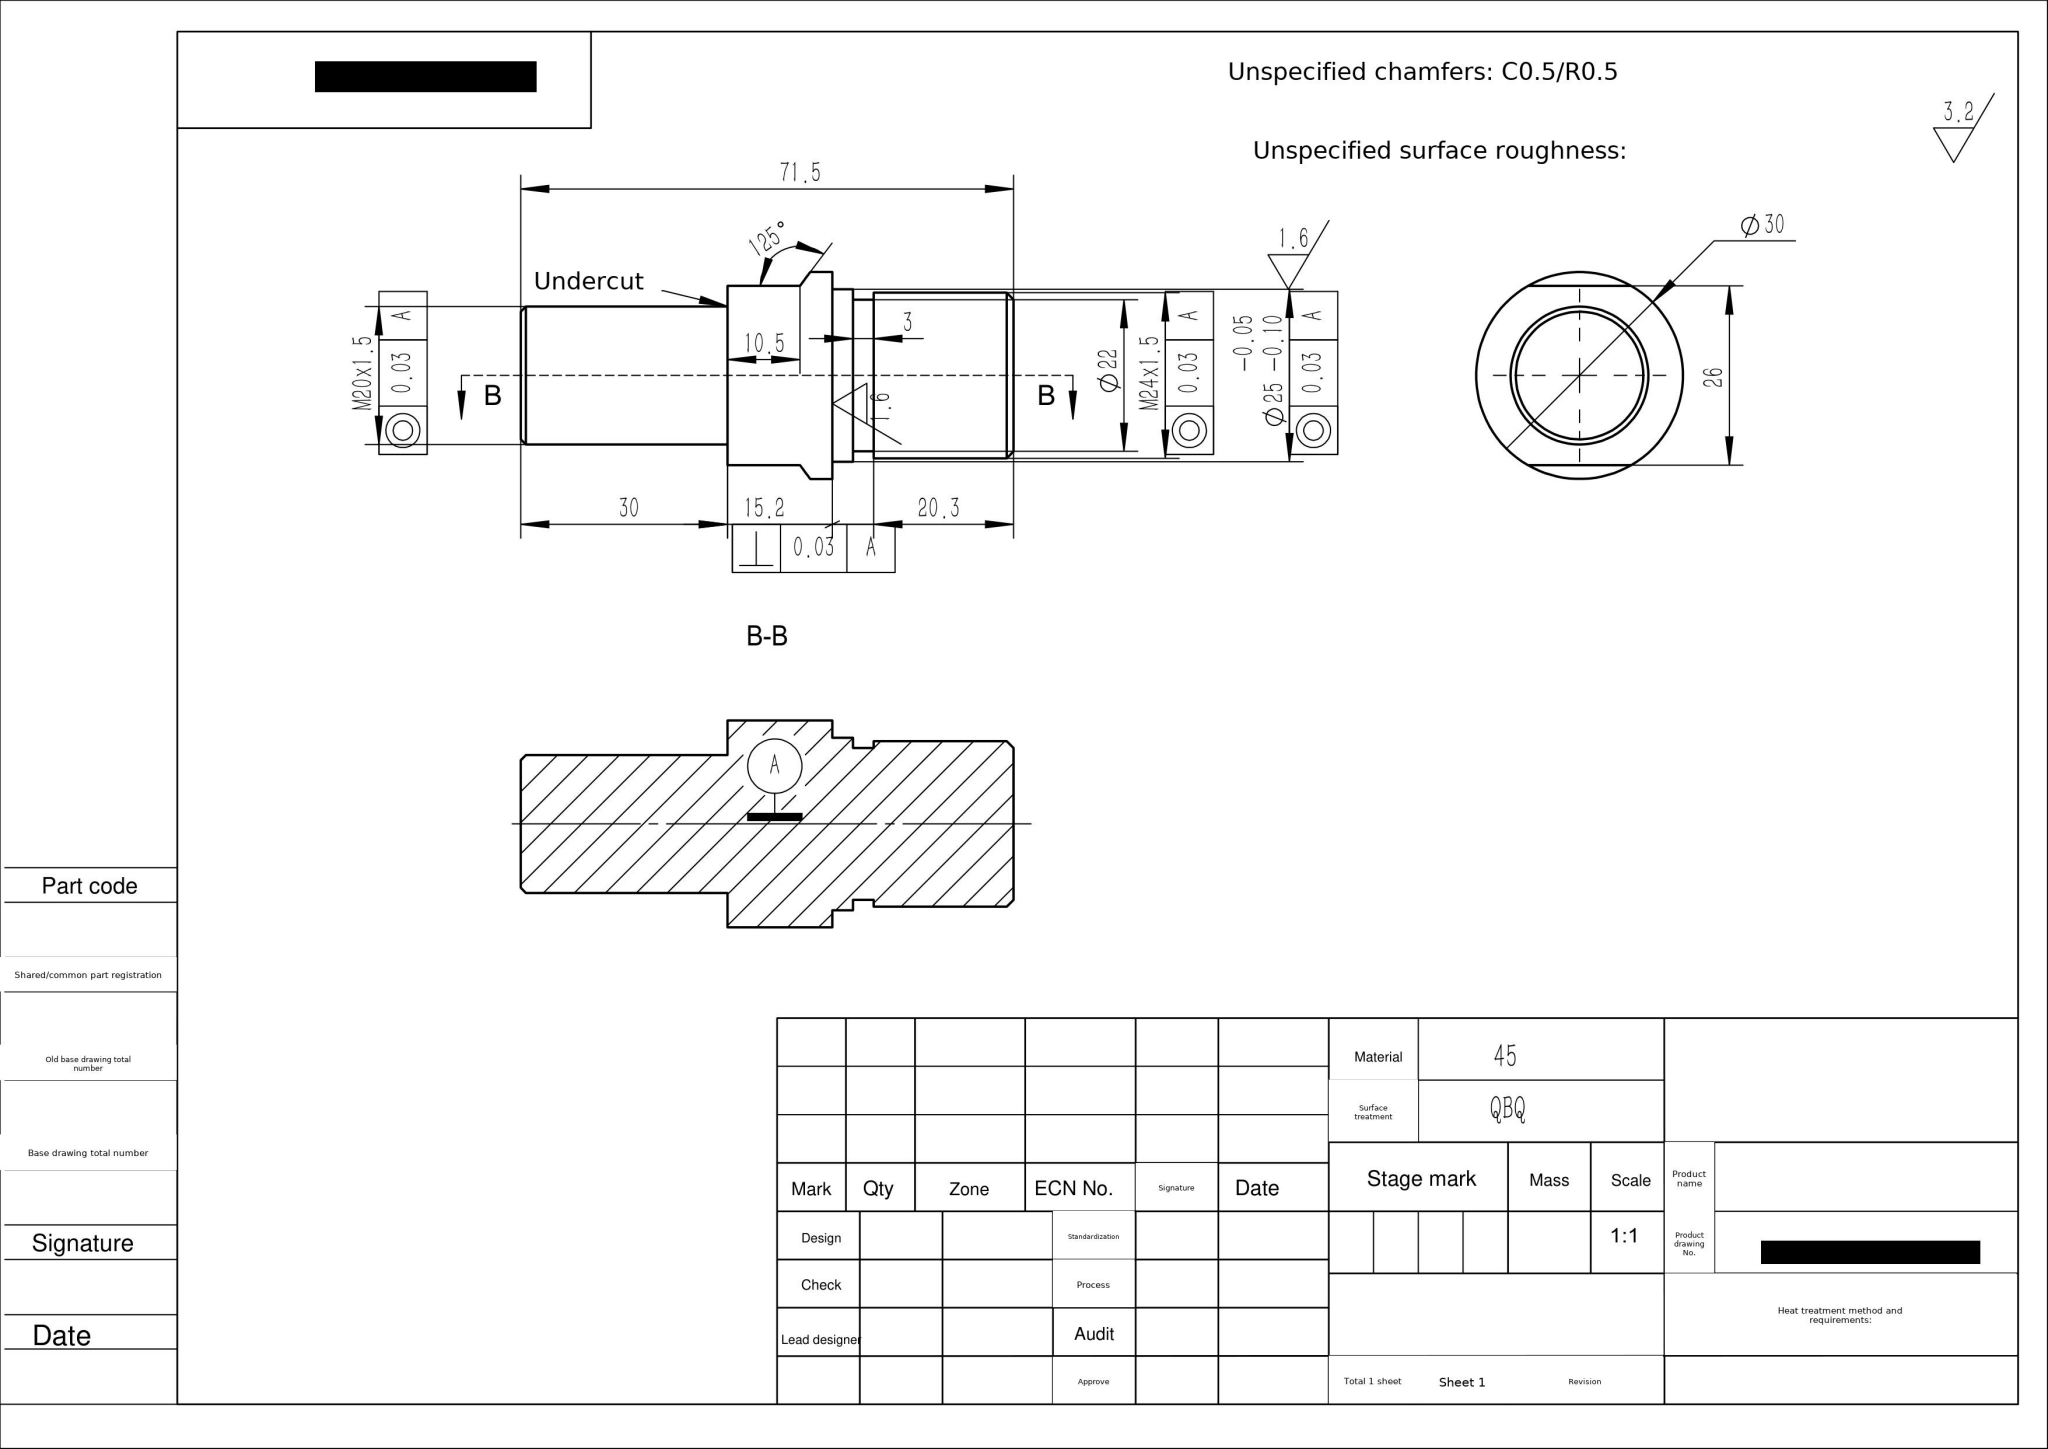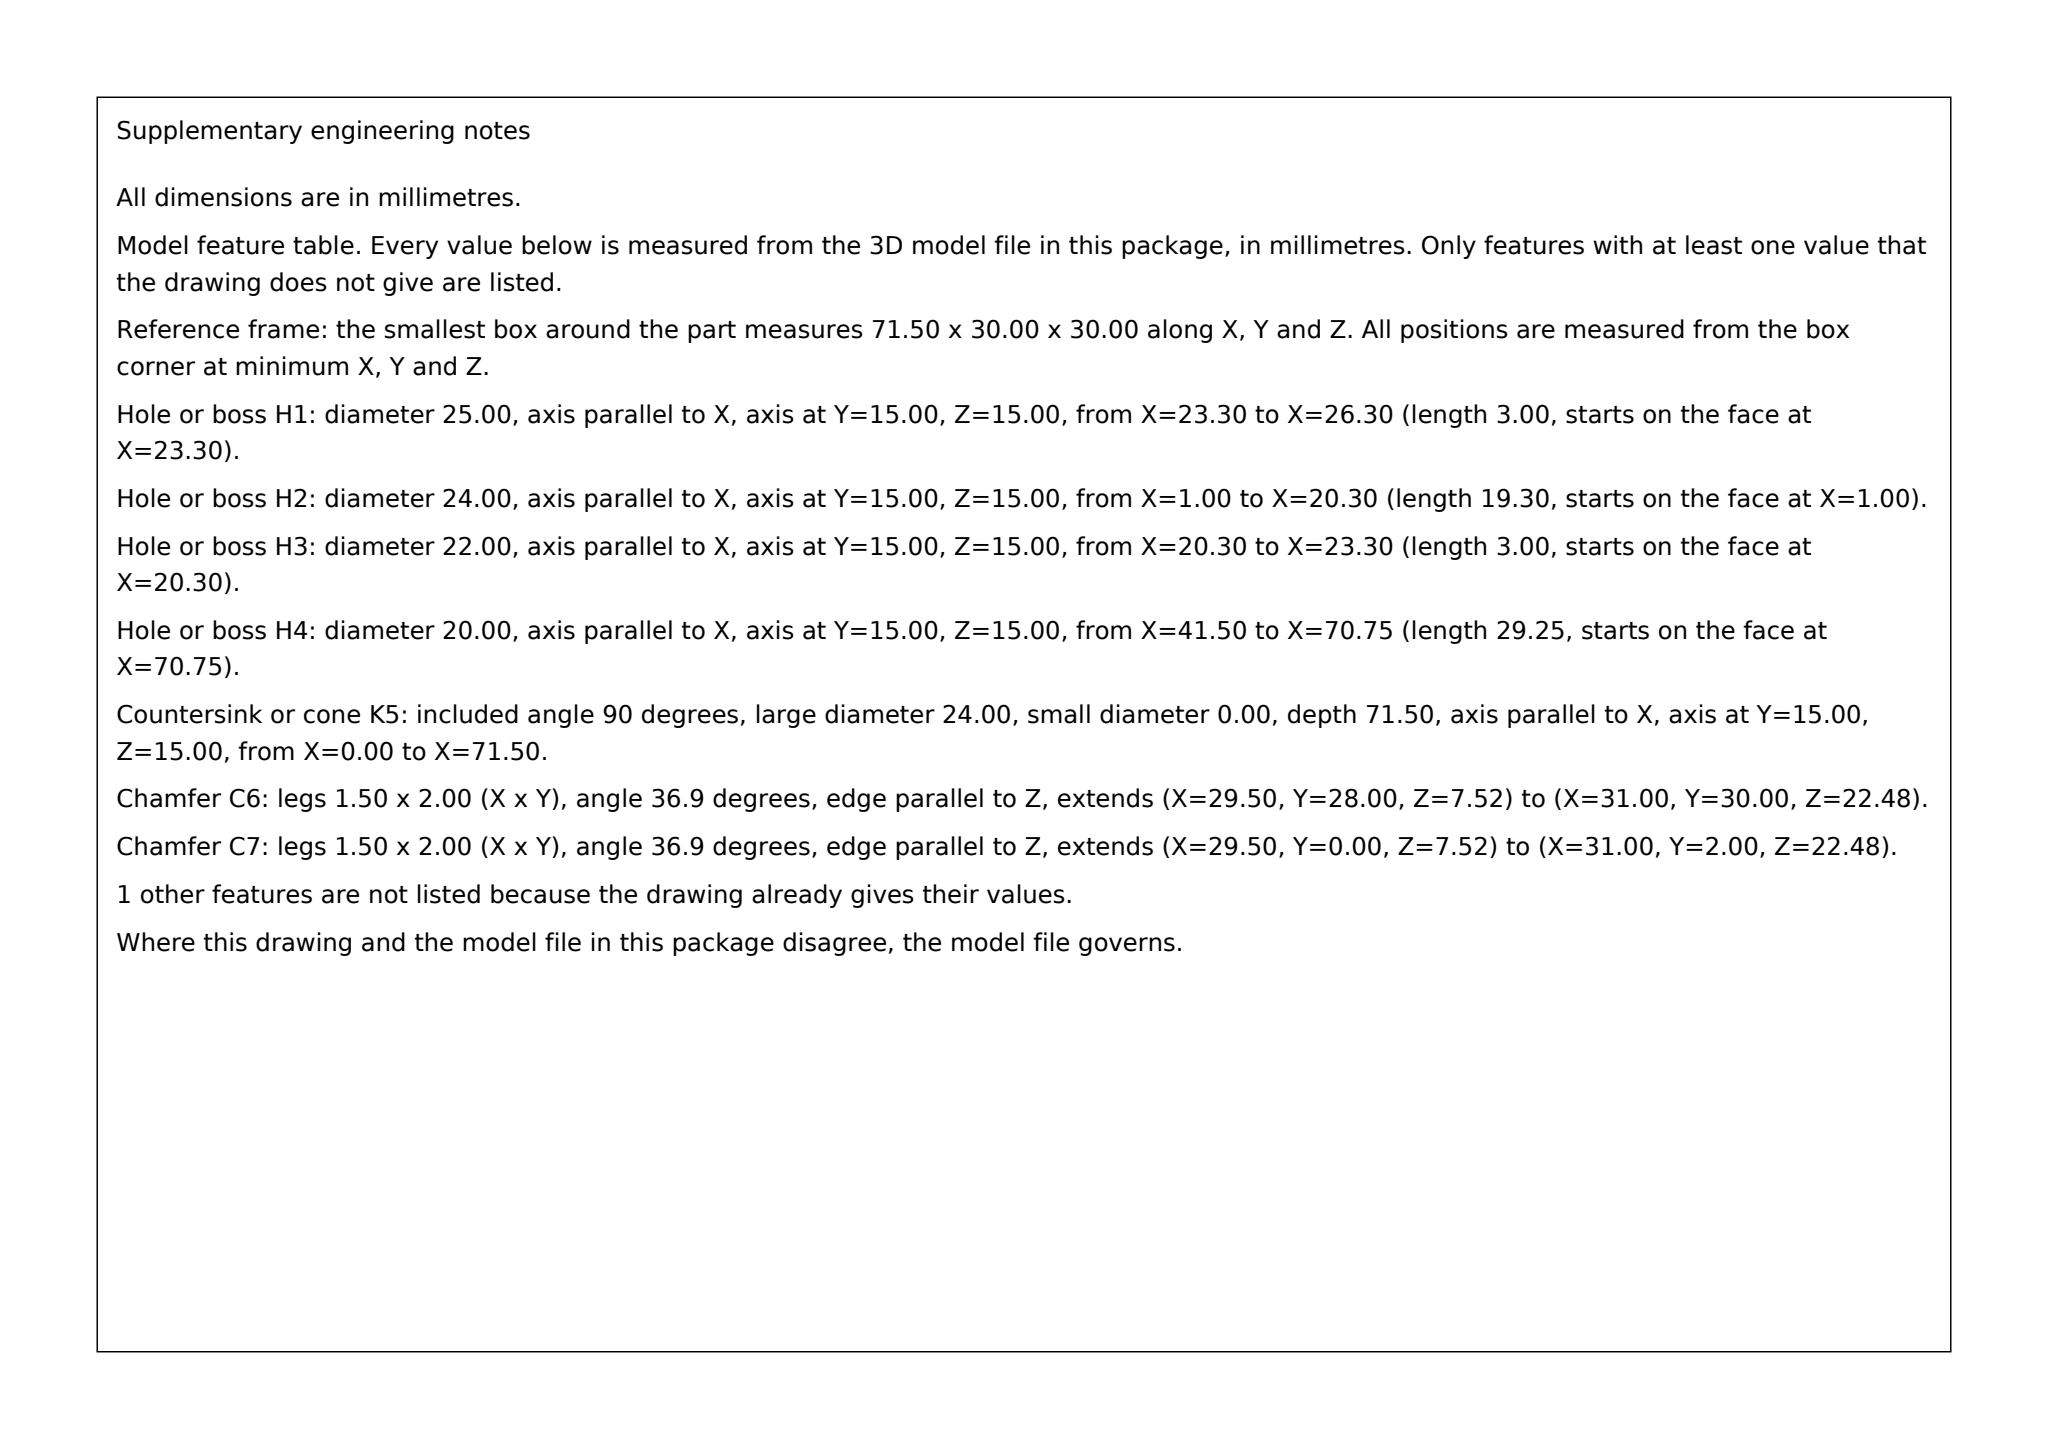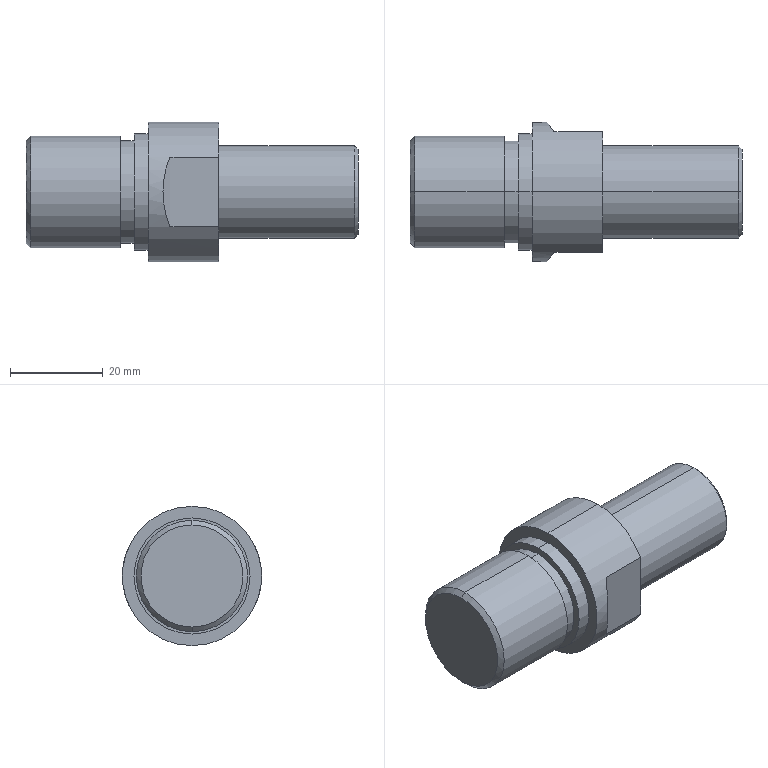Part | SolidWorks | mm | material 45 | 1 solid | 24 faces | box 71.5 x 30 x 30 mm | volume 31462 mm3 | cylinder 10 | plane 10 | cone 4 | commonest cylinder face diameters 20 x2 24 x2 22 x2 25 x2 30 x2
STEP:
#1=CARTESIAN_POINT('',(35.75,0.,-9.25));
#2=VERTEX_POINT('',#1);
#3=CARTESIAN_POINT('',(35.75,0.,9.25));
#4=VERTEX_POINT('',#3);
#5=CARTESIAN_POINT('',(35.75,0.,0.));
#6=DIRECTION('',(1.,0.,0.));
#7=DIRECTION('',(0.,0.,-1.));
#8=AXIS2_PLACEMENT_3D('',#5,#6,#7);
#9=CIRCLE('',#8,9.25);
#10=EDGE_CURVE('',#2,#4,#9,.T.);
#11=ORIENTED_EDGE('',*,*,#10,.F.);
#12=CARTESIAN_POINT('',(35.,0.,-10.));
#13=VERTEX_POINT('',#12);
#14=CARTESIAN_POINT('',(35.75,0.,-9.25));
#15=DIRECTION('',(-0.7071,0.,-0.7071));
#16=VECTOR('',#15,1000.);
#17=LINE('',#14,#16);
#18=EDGE_CURVE('',#2,#13,#17,.T.);
#19=ORIENTED_EDGE('',*,*,#18,.T.);
#20=CARTESIAN_POINT('',(35.,0.,10.));
#21=VERTEX_POINT('',#20);
#22=CARTESIAN_POINT('',(35.,0.,0.));
#23=DIRECTION('',(-1.,0.,0.));
#24=DIRECTION('',(0.,0.,-1.));
#25=AXIS2_PLACEMENT_3D('',#22,#23,#24);
#26=CIRCLE('',#25,10.);
#27=EDGE_CURVE('',#21,#13,#26,.T.);
#28=ORIENTED_EDGE('',*,*,#27,.F.);
#29=CARTESIAN_POINT('',(35.75,0.,9.25));
#30=DIRECTION('',(-0.7071,0.,0.7071));
#31=VECTOR('',#30,1000.);
#32=LINE('',#29,#31);
#33=EDGE_CURVE('',#4,#21,#32,.T.);
#34=ORIENTED_EDGE('',*,*,#33,.F.);
#35=EDGE_LOOP('',(#11,#19,#28,#34));
#36=FACE_OUTER_BOUND('',#35,.T.);
#37=CARTESIAN_POINT('',(35.75,0.,0.));
#38=DIRECTION('',(-1.,0.,0.));
#39=DIRECTION('',(0.,0.,1.));
#40=AXIS2_PLACEMENT_3D('',#37,#38,#39);
#41=CONICAL_SURFACE('',#40,9.25,0.7854);
#42=ADVANCED_FACE('',(#36),#41,.T.);
#43=ORIENTED_EDGE('',*,*,#27,.T.);
#44=CARTESIAN_POINT('',(5.75,0.,-10.));
#45=VERTEX_POINT('',#44);
#46=CARTESIAN_POINT('',(48.75,0.,-10.));
#47=DIRECTION('',(-1.,0.,0.));
#48=VECTOR('',#47,1000.);
#49=LINE('',#46,#48);
#50=EDGE_CURVE('',#13,#45,#49,.T.);
#51=ORIENTED_EDGE('',*,*,#50,.T.);
#52=CARTESIAN_POINT('',(5.75,0.,10.));
#53=VERTEX_POINT('',#52);
#54=CARTESIAN_POINT('',(5.75,0.,0.));
#55=DIRECTION('',(1.,0.,0.));
#56=DIRECTION('',(0.,0.,-1.));
#57=AXIS2_PLACEMENT_3D('',#54,#55,#56);
#58=CIRCLE('',#57,10.);
#59=EDGE_CURVE('',#45,#53,#58,.T.);
#60=ORIENTED_EDGE('',*,*,#59,.T.);
#61=CARTESIAN_POINT('',(48.75,0.,10.));
#62=DIRECTION('',(-1.,0.,0.));
#63=VECTOR('',#62,1000.);
#64=LINE('',#61,#63);
#65=EDGE_CURVE('',#21,#53,#64,.T.);
#66=ORIENTED_EDGE('',*,*,#65,.F.);
#67=EDGE_LOOP('',(#43,#51,#60,#66));
#68=FACE_OUTER_BOUND('',#67,.T.);
#69=CARTESIAN_POINT('',(48.75,0.,0.));
#70=DIRECTION('',(-1.,0.,0.));
#71=DIRECTION('',(0.,0.,1.));
#72=AXIS2_PLACEMENT_3D('',#69,#70,#71);
#73=CYLINDRICAL_SURFACE('',#72,10.);
#74=ADVANCED_FACE('',(#68),#73,.T.);
#75=CARTESIAN_POINT('',(-15.45,0.,-12.));
#76=VERTEX_POINT('',#75);
#77=CARTESIAN_POINT('',(-15.45,0.,12.));
#78=VERTEX_POINT('',#77);
#79=CARTESIAN_POINT('',(-15.45,0.,0.));
#80=DIRECTION('',(1.,0.,0.));
#81=DIRECTION('',(0.,0.,1.));
#82=AXIS2_PLACEMENT_3D('',#79,#80,#81);
#83=CIRCLE('',#82,12.);
#84=EDGE_CURVE('',#76,#78,#83,.T.);
#85=ORIENTED_EDGE('',*,*,#84,.F.);
#86=CARTESIAN_POINT('',(-34.75,0.,-12.));
#87=VERTEX_POINT('',#86);
#88=CARTESIAN_POINT('',(-11.75,0.,-12.));
#89=DIRECTION('',(-1.,0.,0.));
#90=VECTOR('',#89,1000.);
#91=LINE('',#88,#90);
#92=EDGE_CURVE('',#76,#87,#91,.T.);
#93=ORIENTED_EDGE('',*,*,#92,.T.);
#94=CARTESIAN_POINT('',(-34.75,0.,12.));
#95=VERTEX_POINT('',#94);
#96=CARTESIAN_POINT('',(-34.75,0.,0.));
#97=DIRECTION('',(1.,0.,0.));
#98=DIRECTION('',(0.,0.,1.));
#99=AXIS2_PLACEMENT_3D('',#96,#97,#98);
#100=CIRCLE('',#99,12.);
#101=EDGE_CURVE('',#87,#95,#100,.T.);
#102=ORIENTED_EDGE('',*,*,#101,.T.);
#103=CARTESIAN_POINT('',(-11.75,0.,12.));
#104=DIRECTION('',(-1.,0.,0.));
#105=VECTOR('',#104,1000.);
#106=LINE('',#103,#105);
#107=EDGE_CURVE('',#78,#95,#106,.T.);
#108=ORIENTED_EDGE('',*,*,#107,.F.);
#109=EDGE_LOOP('',(#85,#93,#102,#108));
#110=FACE_OUTER_BOUND('',#109,.T.);
#111=CARTESIAN_POINT('',(-11.75,0.,0.));
#112=DIRECTION('',(-1.,0.,0.));
#113=DIRECTION('',(0.,0.,1.));
#114=AXIS2_PLACEMENT_3D('',#111,#112,#113);
#115=CYLINDRICAL_SURFACE('',#114,12.);
#116=ADVANCED_FACE('',(#110),#115,.T.);
#117=CARTESIAN_POINT('',(-35.75,0.,-11.));
#118=VERTEX_POINT('',#117);
#119=CARTESIAN_POINT('',(-35.75,0.,11.));
#120=VERTEX_POINT('',#119);
#121=CARTESIAN_POINT('',(-35.75,0.,0.));
#122=DIRECTION('',(1.,0.,0.));
#123=DIRECTION('',(0.,0.,-1.));
#124=AXIS2_PLACEMENT_3D('',#121,#122,#123);
#125=CIRCLE('',#124,11.);
#126=EDGE_CURVE('',#118,#120,#125,.T.);
#127=ORIENTED_EDGE('',*,*,#126,.T.);
#128=CARTESIAN_POINT('',(-34.75,0.,12.));
#129=DIRECTION('',(0.7071,0.,0.7071));
#130=VECTOR('',#129,1000.);
#131=LINE('',#128,#130);
#132=EDGE_CURVE('',#120,#95,#131,.T.);
#133=ORIENTED_EDGE('',*,*,#132,.T.);
#134=ORIENTED_EDGE('',*,*,#101,.F.);
#135=CARTESIAN_POINT('',(-34.75,0.,-12.));
#136=DIRECTION('',(0.7071,0.,-0.7071));
#137=VECTOR('',#136,1000.);
#138=LINE('',#135,#137);
#139=EDGE_CURVE('',#118,#87,#138,.T.);
#140=ORIENTED_EDGE('',*,*,#139,.F.);
#141=EDGE_LOOP('',(#127,#133,#134,#140));
#142=FACE_OUTER_BOUND('',#141,.T.);
#143=CARTESIAN_POINT('',(-34.75,0.,0.));
#144=DIRECTION('',(1.,0.,0.));
#145=DIRECTION('',(0.,0.,-1.));
#146=AXIS2_PLACEMENT_3D('',#143,#144,#145);
#147=CONICAL_SURFACE('',#146,12.,0.7854);
#148=ADVANCED_FACE('',(#142),#147,.T.);
#149=CARTESIAN_POINT('',(-15.45,0.,11.));
#150=VERTEX_POINT('',#149);
#151=CARTESIAN_POINT('',(-15.45,0.,-11.));
#152=VERTEX_POINT('',#151);
#153=CARTESIAN_POINT('',(-15.45,0.,0.));
#154=DIRECTION('',(-1.,0.,0.));
#155=DIRECTION('',(0.,0.,1.));
#156=AXIS2_PLACEMENT_3D('',#153,#154,#155);
#157=CIRCLE('',#156,11.);
#158=EDGE_CURVE('',#150,#152,#157,.T.);
#159=ORIENTED_EDGE('',*,*,#158,.F.);
#160=CARTESIAN_POINT('',(-12.45,0.,11.));
#161=VERTEX_POINT('',#160);
#162=CARTESIAN_POINT('',(-15.45,0.,11.));
#163=DIRECTION('',(1.,0.,0.));
#164=VECTOR('',#163,1000.);
#165=LINE('',#162,#164);
#166=EDGE_CURVE('',#150,#161,#165,.T.);
#167=ORIENTED_EDGE('',*,*,#166,.T.);
#168=CARTESIAN_POINT('',(-12.45,0.,-11.));
#169=VERTEX_POINT('',#168);
#170=CARTESIAN_POINT('',(-12.45,0.,0.));
#171=DIRECTION('',(-1.,0.,0.));
#172=DIRECTION('',(0.,0.,1.));
#173=AXIS2_PLACEMENT_3D('',#170,#171,#172);
#174=CIRCLE('',#173,11.);
#175=EDGE_CURVE('',#161,#169,#174,.T.);
#176=ORIENTED_EDGE('',*,*,#175,.T.);
#177=CARTESIAN_POINT('',(-15.45,0.,-11.));
#178=DIRECTION('',(1.,0.,0.));
#179=VECTOR('',#178,1000.);
#180=LINE('',#177,#179);
#181=EDGE_CURVE('',#152,#169,#180,.T.);
#182=ORIENTED_EDGE('',*,*,#181,.F.);
#183=EDGE_LOOP('',(#159,#167,#176,#182));
#184=FACE_OUTER_BOUND('',#183,.T.);
#185=CARTESIAN_POINT('',(-15.45,0.,0.));
#186=DIRECTION('',(1.,0.,0.));
#187=DIRECTION('',(0.,0.,-1.));
#188=AXIS2_PLACEMENT_3D('',#185,#186,#187);
#189=CYLINDRICAL_SURFACE('',#188,11.);
#190=ADVANCED_FACE('',(#184),#189,.T.);
#191=CARTESIAN_POINT('',(-12.45,0.,12.5));
#192=VERTEX_POINT('',#191);
#193=CARTESIAN_POINT('',(-12.45,0.,-12.5));
#194=VERTEX_POINT('',#193);
#195=CARTESIAN_POINT('',(-12.45,0.,0.));
#196=DIRECTION('',(-1.,0.,0.));
#197=DIRECTION('',(0.,0.,1.));
#198=AXIS2_PLACEMENT_3D('',#195,#196,#197);
#199=CIRCLE('',#198,12.5);
#200=EDGE_CURVE('',#192,#194,#199,.T.);
#201=ORIENTED_EDGE('',*,*,#200,.F.);
#202=CARTESIAN_POINT('',(-9.45,0.,12.5));
#203=VERTEX_POINT('',#202);
#204=CARTESIAN_POINT('',(-35.75,0.,12.5));
#205=DIRECTION('',(1.,0.,0.));
#206=VECTOR('',#205,1000.);
#207=LINE('',#204,#206);
#208=EDGE_CURVE('',#192,#203,#207,.T.);
#209=ORIENTED_EDGE('',*,*,#208,.T.);
#210=CARTESIAN_POINT('',(-9.45,0.,-12.5));
#211=VERTEX_POINT('',#210);
#212=CARTESIAN_POINT('',(-9.45,0.,0.));
#213=DIRECTION('',(1.,0.,0.));
#214=DIRECTION('',(0.,0.,1.));
#215=AXIS2_PLACEMENT_3D('',#212,#213,#214);
#216=CIRCLE('',#215,12.5);
#217=EDGE_CURVE('',#211,#203,#216,.T.);
#218=ORIENTED_EDGE('',*,*,#217,.F.);
#219=CARTESIAN_POINT('',(-35.75,0.,-12.5));
#220=DIRECTION('',(1.,0.,0.));
#221=VECTOR('',#220,1000.);
#222=LINE('',#219,#221);
#223=EDGE_CURVE('',#194,#211,#222,.T.);
#224=ORIENTED_EDGE('',*,*,#223,.F.);
#225=EDGE_LOOP('',(#201,#209,#218,#224));
#226=FACE_OUTER_BOUND('',#225,.T.);
#227=CARTESIAN_POINT('',(-35.75,0.,0.));
#228=DIRECTION('',(1.,0.,0.));
#229=DIRECTION('',(0.,0.,-1.));
#230=AXIS2_PLACEMENT_3D('',#227,#228,#229);
#231=CYLINDRICAL_SURFACE('',#230,12.5);
#232=ADVANCED_FACE('',(#226),#231,.T.);
#233=CARTESIAN_POINT('',(5.75,0.,-15.));
#234=VERTEX_POINT('',#233);
#235=CARTESIAN_POINT('',(5.75,13.,-7.483));
#236=VERTEX_POINT('',#235);
#237=CARTESIAN_POINT('',(5.75,0.,0.));
#238=DIRECTION('',(1.,0.,0.));
#239=DIRECTION('',(0.,0.,1.));
#240=AXIS2_PLACEMENT_3D('',#237,#238,#239);
#241=CIRCLE('',#240,15.);
#242=EDGE_CURVE('',#234,#236,#241,.T.);
#243=ORIENTED_EDGE('',*,*,#242,.F.);
#244=CARTESIAN_POINT('',(-9.45,0.,-15.));
#245=VERTEX_POINT('',#244);
#246=CARTESIAN_POINT('',(8.75,0.,-15.));
#247=DIRECTION('',(-1.,0.,0.));
#248=VECTOR('',#247,1000.);
#249=LINE('',#246,#248);
#250=EDGE_CURVE('',#234,#245,#249,.T.);
#251=ORIENTED_EDGE('',*,*,#250,.T.);
#252=CARTESIAN_POINT('',(-9.45,0.,15.));
#253=VERTEX_POINT('',#252);
#254=CARTESIAN_POINT('',(-9.45,0.,0.));
#255=DIRECTION('',(-1.,0.,0.));
#256=DIRECTION('',(0.,0.,1.));
#257=AXIS2_PLACEMENT_3D('',#254,#255,#256);
#258=CIRCLE('',#257,15.);
#259=EDGE_CURVE('',#253,#245,#258,.T.);
#260=ORIENTED_EDGE('',*,*,#259,.F.);
#261=CARTESIAN_POINT('',(5.75,0.,15.));
#262=VERTEX_POINT('',#261);
#263=CARTESIAN_POINT('',(8.75,0.,15.));
#264=DIRECTION('',(-1.,0.,0.));
#265=VECTOR('',#264,1000.);
#266=LINE('',#263,#265);
#267=EDGE_CURVE('',#262,#253,#266,.T.);
#268=ORIENTED_EDGE('',*,*,#267,.F.);
#269=CARTESIAN_POINT('',(5.75,13.,7.483));
#270=VERTEX_POINT('',#269);
#271=CARTESIAN_POINT('',(5.75,0.,0.));
#272=DIRECTION('',(1.,0.,0.));
#273=DIRECTION('',(0.,0.,1.));
#274=AXIS2_PLACEMENT_3D('',#271,#272,#273);
#275=CIRCLE('',#274,15.);
#276=EDGE_CURVE('',#270,#262,#275,.T.);
#277=ORIENTED_EDGE('',*,*,#276,.F.);
#278=CARTESIAN_POINT('',(-4.75,13.,7.483));
#279=VERTEX_POINT('',#278);
#280=CARTESIAN_POINT('',(-4.75,13.,7.483));
#281=DIRECTION('',(1.,0.,0.));
#282=VECTOR('',#281,1000.);
#283=LINE('',#280,#282);
#284=EDGE_CURVE('',#279,#270,#283,.T.);
#285=ORIENTED_EDGE('',*,*,#284,.F.);
#286=CARTESIAN_POINT('',(-4.75,13.,-7.483));
#287=VERTEX_POINT('',#286);
#288=CARTESIAN_POINT('',(-4.75,13.,7.483));
#289=CARTESIAN_POINT('',(-6.799,15.732,2.738));
#290=CARTESIAN_POINT('',(-6.799,15.732,-2.738));
#291=CARTESIAN_POINT('',(-4.75,13.,-7.483));
#292=(BOUNDED_CURVE()B_SPLINE_CURVE(3,(#288,#289,#290,#291),.UNSPECIFIED.,.F.,.T.)B_SPLINE_CURVE_WITH_KNOTS((4,4),(5.761,6.806),.UNSPECIFIED.)CURVE()GEOMETRIC_REPRESENTATION_ITEM()RATIONAL_B_SPLINE_CURVE((1.,0.9111,0.9111,1.))REPRESENTATION_ITEM(''));
#293=EDGE_CURVE('',#279,#287,#292,.T.);
#294=ORIENTED_EDGE('',*,*,#293,.T.);
#295=CARTESIAN_POINT('',(-4.75,13.,-7.483));
#296=DIRECTION('',(-1.,0.,0.));
#297=VECTOR('',#296,1000.);
#298=LINE('',#295,#297);
#299=EDGE_CURVE('',#236,#287,#298,.T.);
#300=ORIENTED_EDGE('',*,*,#299,.F.);
#301=EDGE_LOOP('',(#243,#251,#260,#268,#277,#285,#294,#300));
#302=FACE_OUTER_BOUND('',#301,.T.);
#303=CARTESIAN_POINT('',(8.75,0.,0.));
#304=DIRECTION('',(-1.,0.,0.));
#305=DIRECTION('',(0.,0.,1.));
#306=AXIS2_PLACEMENT_3D('',#303,#304,#305);
#307=CYLINDRICAL_SURFACE('',#306,15.);
#308=ADVANCED_FACE('',(#302),#307,.T.);
#309=CARTESIAN_POINT('',(5.75,0.,0.));
#310=DIRECTION('',(1.,0.,0.));
#311=DIRECTION('',(0.,0.,-1.));
#312=AXIS2_PLACEMENT_3D('',#309,#310,#311);
#313=CIRCLE('',#312,10.);
#314=EDGE_CURVE('',#53,#45,#313,.T.);
#315=ORIENTED_EDGE('',*,*,#314,.F.);
#316=ORIENTED_EDGE('',*,*,#59,.F.);
#317=EDGE_LOOP('',(#315,#316));
#318=FACE_BOUND('',#317,.T.);
#319=CARTESIAN_POINT('',(5.75,-13.,-7.483));
#320=VERTEX_POINT('',#319);
#321=CARTESIAN_POINT('',(5.75,0.,0.));
#322=DIRECTION('',(1.,0.,0.));
#323=DIRECTION('',(0.,0.,1.));
#324=AXIS2_PLACEMENT_3D('',#321,#322,#323);
#325=CIRCLE('',#324,15.);
#326=EDGE_CURVE('',#320,#234,#325,.T.);
#327=ORIENTED_EDGE('',*,*,#326,.T.);
#328=ORIENTED_EDGE('',*,*,#242,.T.);
#329=CARTESIAN_POINT('',(5.75,13.,0.));
#330=DIRECTION('',(0.,0.,1.));
#331=VECTOR('',#330,1000.);
#332=LINE('',#329,#331);
#333=EDGE_CURVE('',#236,#270,#332,.T.);
#334=ORIENTED_EDGE('',*,*,#333,.T.);
#335=ORIENTED_EDGE('',*,*,#276,.T.);
#336=CARTESIAN_POINT('',(5.75,-13.,7.483));
#337=VERTEX_POINT('',#336);
#338=CARTESIAN_POINT('',(5.75,0.,0.));
#339=DIRECTION('',(1.,0.,0.));
#340=DIRECTION('',(0.,0.,1.));
#341=AXIS2_PLACEMENT_3D('',#338,#339,#340);
#342=CIRCLE('',#341,15.);
#343=EDGE_CURVE('',#262,#337,#342,.T.);
#344=ORIENTED_EDGE('',*,*,#343,.T.);
#345=CARTESIAN_POINT('',(5.75,-13.,0.));
#346=DIRECTION('',(0.,0.,-1.));
#347=VECTOR('',#346,1000.);
#348=LINE('',#345,#347);
#349=EDGE_CURVE('',#337,#320,#348,.T.);
#350=ORIENTED_EDGE('',*,*,#349,.T.);
#351=EDGE_LOOP('',(#327,#328,#334,#335,#344,#350));
#352=FACE_OUTER_BOUND('',#351,.T.);
#353=CARTESIAN_POINT('',(5.75,0.,0.));
#354=DIRECTION('',(1.,0.,0.));
#355=DIRECTION('',(0.,0.,-1.));
#356=AXIS2_PLACEMENT_3D('',#353,#354,#355);
#357=PLANE('',#356);
#358=ADVANCED_FACE('',(#318,#352),#357,.T.);
#359=ORIENTED_EDGE('',*,*,#284,.T.);
#360=ORIENTED_EDGE('',*,*,#333,.F.);
#361=ORIENTED_EDGE('',*,*,#299,.T.);
#362=CARTESIAN_POINT('',(-4.75,13.,21.671));
#363=DIRECTION('',(0.,0.,1.));
#364=VECTOR('',#363,1000.);
#365=LINE('',#362,#364);
#366=EDGE_CURVE('',#287,#279,#365,.T.);
#367=ORIENTED_EDGE('',*,*,#366,.T.);
#368=EDGE_LOOP('',(#359,#360,#361,#367));
#369=FACE_OUTER_BOUND('',#368,.T.);
#370=CARTESIAN_POINT('',(-4.75,13.,21.671));
#371=DIRECTION('',(0.,1.,0.));
#372=DIRECTION('',(0.,0.,1.));
#373=AXIS2_PLACEMENT_3D('',#370,#371,#372);
#374=PLANE('',#373);
#375=ADVANCED_FACE('',(#369),#374,.T.);
#376=ORIENTED_EDGE('',*,*,#250,.F.);
#377=ORIENTED_EDGE('',*,*,#326,.F.);
#378=CARTESIAN_POINT('',(-4.75,-13.,-7.483));
#379=VERTEX_POINT('',#378);
#380=CARTESIAN_POINT('',(8.75,-13.,-7.483));
#381=DIRECTION('',(-1.,0.,0.));
#382=VECTOR('',#381,1000.);
#383=LINE('',#380,#382);
#384=EDGE_CURVE('',#320,#379,#383,.T.);
#385=ORIENTED_EDGE('',*,*,#384,.T.);
#386=CARTESIAN_POINT('',(-4.75,-13.,7.483));
#387=VERTEX_POINT('',#386);
#388=CARTESIAN_POINT('',(-4.75,-13.,-7.483));
#389=CARTESIAN_POINT('',(-6.799,-15.732,-2.738));
#390=CARTESIAN_POINT('',(-6.799,-15.732,2.738));
#391=CARTESIAN_POINT('',(-4.75,-13.,7.483));
#392=(BOUNDED_CURVE()B_SPLINE_CURVE(3,(#388,#389,#390,#391),.UNSPECIFIED.,.F.,.F.)B_SPLINE_CURVE_WITH_KNOTS((4,4),(5.761,6.806),.UNSPECIFIED.)CURVE()GEOMETRIC_REPRESENTATION_ITEM()RATIONAL_B_SPLINE_CURVE((1.,0.9111,0.9111,1.))REPRESENTATION_ITEM(''));
#393=EDGE_CURVE('',#379,#387,#392,.T.);
#394=ORIENTED_EDGE('',*,*,#393,.T.);
#395=CARTESIAN_POINT('',(8.75,-13.,7.483));
#396=DIRECTION('',(1.,0.,0.));
#397=VECTOR('',#396,1000.);
#398=LINE('',#395,#397);
#399=EDGE_CURVE('',#387,#337,#398,.T.);
#400=ORIENTED_EDGE('',*,*,#399,.T.);
#401=ORIENTED_EDGE('',*,*,#343,.F.);
#402=ORIENTED_EDGE('',*,*,#267,.T.);
#403=CARTESIAN_POINT('',(-9.45,0.,0.));
#404=DIRECTION('',(-1.,0.,0.));
#405=DIRECTION('',(0.,0.,1.));
#406=AXIS2_PLACEMENT_3D('',#403,#404,#405);
#407=CIRCLE('',#406,15.);
#408=EDGE_CURVE('',#245,#253,#407,.T.);
#409=ORIENTED_EDGE('',*,*,#408,.F.);
#410=EDGE_LOOP('',(#376,#377,#385,#394,#400,#401,#402,#409));
#411=FACE_OUTER_BOUND('',#410,.T.);
#412=CARTESIAN_POINT('',(8.75,0.,0.));
#413=DIRECTION('',(-1.,0.,0.));
#414=DIRECTION('',(0.,0.,1.));
#415=AXIS2_PLACEMENT_3D('',#412,#413,#414);
#416=CYLINDRICAL_SURFACE('',#415,15.);
#417=ADVANCED_FACE('',(#411),#416,.T.);
#418=ORIENTED_EDGE('',*,*,#384,.F.);
#419=ORIENTED_EDGE('',*,*,#349,.F.);
#420=ORIENTED_EDGE('',*,*,#399,.F.);
#421=CARTESIAN_POINT('',(-4.75,-13.,21.671));
#422=DIRECTION('',(0.,0.,-1.));
#423=VECTOR('',#422,1000.);
#424=LINE('',#421,#423);
#425=EDGE_CURVE('',#387,#379,#424,.T.);
#426=ORIENTED_EDGE('',*,*,#425,.T.);
#427=EDGE_LOOP('',(#418,#419,#420,#426));
#428=FACE_OUTER_BOUND('',#427,.T.);
#429=CARTESIAN_POINT('',(-4.75,-13.,21.671));
#430=DIRECTION('',(0.,-1.,0.));
#431=DIRECTION('',(0.,0.,-1.));
#432=AXIS2_PLACEMENT_3D('',#429,#430,#431);
#433=PLANE('',#432);
#434=ADVANCED_FACE('',(#428),#433,.T.);
#435=ORIENTED_EDGE('',*,*,#366,.F.);
#436=ORIENTED_EDGE('',*,*,#293,.F.);
#437=EDGE_LOOP('',(#435,#436));
#438=FACE_OUTER_BOUND('',#437,.T.);
#439=CARTESIAN_POINT('',(-4.75,13.,-15.));
#440=DIRECTION('',(-0.8,-0.6,0.));
#441=DIRECTION('',(0.6,-0.8,0.));
#442=AXIS2_PLACEMENT_3D('',#439,#440,#441);
#443=PLANE('',#442);
#444=ADVANCED_FACE('',(#438),#443,.F.);
#445=ORIENTED_EDGE('',*,*,#393,.F.);
#446=ORIENTED_EDGE('',*,*,#425,.F.);
#447=EDGE_LOOP('',(#445,#446));
#448=FACE_OUTER_BOUND('',#447,.T.);
#449=CARTESIAN_POINT('',(-4.75,-13.,-15.));
#450=DIRECTION('',(0.8,-0.6,0.));
#451=DIRECTION('',(0.6,0.8,0.));
#452=AXIS2_PLACEMENT_3D('',#449,#450,#451);
#453=PLANE('',#452);
#454=ADVANCED_FACE('',(#448),#453,.T.);
#455=ORIENTED_EDGE('',*,*,#259,.T.);
#456=ORIENTED_EDGE('',*,*,#408,.T.);
#457=EDGE_LOOP('',(#455,#456));
#458=FACE_OUTER_BOUND('',#457,.T.);
#459=ORIENTED_EDGE('',*,*,#217,.T.);
#460=CARTESIAN_POINT('',(-9.45,0.,0.));
#461=DIRECTION('',(1.,0.,0.));
#462=DIRECTION('',(0.,0.,1.));
#463=AXIS2_PLACEMENT_3D('',#460,#461,#462);
#464=CIRCLE('',#463,12.5);
#465=EDGE_CURVE('',#203,#211,#464,.T.);
#466=ORIENTED_EDGE('',*,*,#465,.T.);
#467=EDGE_LOOP('',(#459,#466));
#468=FACE_BOUND('',#467,.T.);
#469=CARTESIAN_POINT('',(-9.45,0.,0.));
#470=DIRECTION('',(-1.,0.,0.));
#471=DIRECTION('',(0.,0.,1.));
#472=AXIS2_PLACEMENT_3D('',#469,#470,#471);
#473=PLANE('',#472);
#474=ADVANCED_FACE('',(#458,#468),#473,.T.);
#475=ORIENTED_EDGE('',*,*,#208,.F.);
#476=CARTESIAN_POINT('',(-12.45,0.,0.));
#477=DIRECTION('',(-1.,0.,0.));
#478=DIRECTION('',(0.,0.,1.));
#479=AXIS2_PLACEMENT_3D('',#476,#477,#478);
#480=CIRCLE('',#479,12.5);
#481=EDGE_CURVE('',#194,#192,#480,.T.);
#482=ORIENTED_EDGE('',*,*,#481,.F.);
#483=ORIENTED_EDGE('',*,*,#223,.T.);
#484=ORIENTED_EDGE('',*,*,#465,.F.);
#485=EDGE_LOOP('',(#475,#482,#483,#484));
#486=FACE_OUTER_BOUND('',#485,.T.);
#487=CARTESIAN_POINT('',(-35.75,0.,0.));
#488=DIRECTION('',(1.,0.,0.));
#489=DIRECTION('',(0.,0.,-1.));
#490=AXIS2_PLACEMENT_3D('',#487,#488,#489);
#491=CYLINDRICAL_SURFACE('',#490,12.5);
#492=ADVANCED_FACE('',(#486),#491,.T.);
#493=ORIENTED_EDGE('',*,*,#481,.T.);
#494=ORIENTED_EDGE('',*,*,#200,.T.);
#495=EDGE_LOOP('',(#493,#494));
#496=FACE_OUTER_BOUND('',#495,.T.);
#497=CARTESIAN_POINT('',(-12.45,0.,0.));
#498=DIRECTION('',(-1.,0.,0.));
#499=DIRECTION('',(0.,0.,1.));
#500=AXIS2_PLACEMENT_3D('',#497,#498,#499);
#501=CIRCLE('',#500,11.);
#502=EDGE_CURVE('',#169,#161,#501,.T.);
#503=ORIENTED_EDGE('',*,*,#502,.F.);
#504=ORIENTED_EDGE('',*,*,#175,.F.);
#505=EDGE_LOOP('',(#503,#504));
#506=FACE_BOUND('',#505,.T.);
#507=CARTESIAN_POINT('',(-12.45,0.,0.));
#508=DIRECTION('',(-1.,0.,0.));
#509=DIRECTION('',(0.,0.,1.));
#510=AXIS2_PLACEMENT_3D('',#507,#508,#509);
#511=PLANE('',#510);
#512=ADVANCED_FACE('',(#496,#506),#511,.T.);
#513=CARTESIAN_POINT('',(-15.45,0.,0.));
#514=DIRECTION('',(1.,0.,0.));
#515=DIRECTION('',(0.,0.,1.));
#516=AXIS2_PLACEMENT_3D('',#513,#514,#515);
#517=CIRCLE('',#516,12.);
#518=EDGE_CURVE('',#78,#76,#517,.T.);
#519=ORIENTED_EDGE('',*,*,#518,.T.);
#520=ORIENTED_EDGE('',*,*,#84,.T.);
#521=EDGE_LOOP('',(#519,#520));
#522=FACE_OUTER_BOUND('',#521,.T.);
#523=CARTESIAN_POINT('',(-15.45,0.,0.));
#524=DIRECTION('',(-1.,0.,0.));
#525=DIRECTION('',(0.,0.,1.));
#526=AXIS2_PLACEMENT_3D('',#523,#524,#525);
#527=CIRCLE('',#526,11.);
#528=EDGE_CURVE('',#152,#150,#527,.T.);
#529=ORIENTED_EDGE('',*,*,#528,.T.);
#530=ORIENTED_EDGE('',*,*,#158,.T.);
#531=EDGE_LOOP('',(#529,#530));
#532=FACE_BOUND('',#531,.T.);
#533=CARTESIAN_POINT('',(-15.45,0.,0.));
#534=DIRECTION('',(-1.,0.,0.));
#535=DIRECTION('',(0.,0.,1.));
#536=AXIS2_PLACEMENT_3D('',#533,#534,#535);
#537=PLANE('',#536);
#538=ADVANCED_FACE('',(#522,#532),#537,.F.);
#539=ORIENTED_EDGE('',*,*,#166,.F.);
#540=ORIENTED_EDGE('',*,*,#528,.F.);
#541=ORIENTED_EDGE('',*,*,#181,.T.);
#542=ORIENTED_EDGE('',*,*,#502,.T.);
#543=EDGE_LOOP('',(#539,#540,#541,#542));
#544=FACE_OUTER_BOUND('',#543,.T.);
#545=CARTESIAN_POINT('',(-15.45,0.,0.));
#546=DIRECTION('',(1.,0.,0.));
#547=DIRECTION('',(0.,0.,-1.));
#548=AXIS2_PLACEMENT_3D('',#545,#546,#547);
#549=CYLINDRICAL_SURFACE('',#548,11.);
#550=ADVANCED_FACE('',(#544),#549,.T.);
#551=ORIENTED_EDGE('',*,*,#126,.F.);
#552=CARTESIAN_POINT('',(-35.75,0.,0.));
#553=DIRECTION('',(1.,0.,0.));
#554=DIRECTION('',(0.,0.,-1.));
#555=AXIS2_PLACEMENT_3D('',#552,#553,#554);
#556=CIRCLE('',#555,11.);
#557=EDGE_CURVE('',#120,#118,#556,.T.);
#558=ORIENTED_EDGE('',*,*,#557,.F.);
#559=EDGE_LOOP('',(#551,#558));
#560=FACE_OUTER_BOUND('',#559,.T.);
#561=CARTESIAN_POINT('',(-35.75,0.,0.));
#562=DIRECTION('',(-1.,0.,0.));
#563=DIRECTION('',(0.,0.,1.));
#564=AXIS2_PLACEMENT_3D('',#561,#562,#563);
#565=PLANE('',#564);
#566=ADVANCED_FACE('',(#560),#565,.T.);
#567=ORIENTED_EDGE('',*,*,#132,.F.);
#568=ORIENTED_EDGE('',*,*,#557,.T.);
#569=ORIENTED_EDGE('',*,*,#139,.T.);
#570=CARTESIAN_POINT('',(-34.75,0.,0.));
#571=DIRECTION('',(1.,0.,0.));
#572=DIRECTION('',(0.,0.,1.));
#573=AXIS2_PLACEMENT_3D('',#570,#571,#572);
#574=CIRCLE('',#573,12.);
#575=EDGE_CURVE('',#95,#87,#574,.T.);
#576=ORIENTED_EDGE('',*,*,#575,.F.);
#577=EDGE_LOOP('',(#567,#568,#569,#576));
#578=FACE_OUTER_BOUND('',#577,.T.);
#579=CARTESIAN_POINT('',(-34.75,0.,0.));
#580=DIRECTION('',(1.,0.,0.));
#581=DIRECTION('',(0.,0.,-1.));
#582=AXIS2_PLACEMENT_3D('',#579,#580,#581);
#583=CONICAL_SURFACE('',#582,12.,0.7854);
#584=ADVANCED_FACE('',(#578),#583,.T.);
#585=ORIENTED_EDGE('',*,*,#92,.F.);
#586=ORIENTED_EDGE('',*,*,#518,.F.);
#587=ORIENTED_EDGE('',*,*,#107,.T.);
#588=ORIENTED_EDGE('',*,*,#575,.T.);
#589=EDGE_LOOP('',(#585,#586,#587,#588));
#590=FACE_OUTER_BOUND('',#589,.T.);
#591=CARTESIAN_POINT('',(-11.75,0.,0.));
#592=DIRECTION('',(-1.,0.,0.));
#593=DIRECTION('',(0.,0.,1.));
#594=AXIS2_PLACEMENT_3D('',#591,#592,#593);
#595=CYLINDRICAL_SURFACE('',#594,12.);
#596=ADVANCED_FACE('',(#590),#595,.T.);
#597=ORIENTED_EDGE('',*,*,#50,.F.);
#598=CARTESIAN_POINT('',(35.,0.,0.));
#599=DIRECTION('',(-1.,0.,0.));
#600=DIRECTION('',(0.,0.,-1.));
#601=AXIS2_PLACEMENT_3D('',#598,#599,#600);
#602=CIRCLE('',#601,10.);
#603=EDGE_CURVE('',#13,#21,#602,.T.);
#604=ORIENTED_EDGE('',*,*,#603,.T.);
#605=ORIENTED_EDGE('',*,*,#65,.T.);
#606=ORIENTED_EDGE('',*,*,#314,.T.);
#607=EDGE_LOOP('',(#597,#604,#605,#606));
#608=FACE_OUTER_BOUND('',#607,.T.);
#609=CARTESIAN_POINT('',(48.75,0.,0.));
#610=DIRECTION('',(-1.,0.,0.));
#611=DIRECTION('',(0.,0.,1.));
#612=AXIS2_PLACEMENT_3D('',#609,#610,#611);
#613=CYLINDRICAL_SURFACE('',#612,10.);
#614=ADVANCED_FACE('',(#608),#613,.T.);
#615=CARTESIAN_POINT('',(35.75,0.,0.));
#616=DIRECTION('',(1.,0.,0.));
#617=DIRECTION('',(0.,0.,-1.));
#618=AXIS2_PLACEMENT_3D('',#615,#616,#617);
#619=CIRCLE('',#618,9.25);
#620=EDGE_CURVE('',#4,#2,#619,.T.);
#621=ORIENTED_EDGE('',*,*,#620,.T.);
#622=ORIENTED_EDGE('',*,*,#10,.T.);
#623=EDGE_LOOP('',(#621,#622));
#624=FACE_OUTER_BOUND('',#623,.T.);
#625=CARTESIAN_POINT('',(35.75,0.,0.));
#626=DIRECTION('',(1.,0.,0.));
#627=DIRECTION('',(0.,0.,-1.));
#628=AXIS2_PLACEMENT_3D('',#625,#626,#627);
#629=PLANE('',#628);
#630=ADVANCED_FACE('',(#624),#629,.T.);
#631=ORIENTED_EDGE('',*,*,#18,.F.);
#632=ORIENTED_EDGE('',*,*,#620,.F.);
#633=ORIENTED_EDGE('',*,*,#33,.T.);
#634=ORIENTED_EDGE('',*,*,#603,.F.);
#635=EDGE_LOOP('',(#631,#632,#633,#634));
#636=FACE_OUTER_BOUND('',#635,.T.);
#637=CARTESIAN_POINT('',(35.75,0.,0.));
#638=DIRECTION('',(-1.,0.,0.));
#639=DIRECTION('',(0.,0.,1.));
#640=AXIS2_PLACEMENT_3D('',#637,#638,#639);
#641=CONICAL_SURFACE('',#640,9.25,0.7854);
#642=ADVANCED_FACE('',(#636),#641,.T.);
#643=CLOSED_SHELL('',(#42,#74,#116,#148,#190,#232,#308,#358,#375,#417,#434,#444,#454,#474,#492,#512,#538,#550,#566,#584,#596,#614,#630,#642));
#644=MANIFOLD_SOLID_BREP('',#643);
#645=CARTESIAN_POINT('',(0.,0.,0.));
#646=DIRECTION('',(0.,0.,1.));
#647=DIRECTION('',(1.,0.,0.));
#648=AXIS2_PLACEMENT_3D('',#645,#646,#647);
#649=(LENGTH_UNIT()NAMED_UNIT(*)SI_UNIT(.MILLI.,.METRE.));
#650=UNCERTAINTY_MEASURE_WITH_UNIT(LENGTH_MEASURE(0.00001),#649,'','');
#651=(NAMED_UNIT(*)PLANE_ANGLE_UNIT()SI_UNIT($,.RADIAN.));
#652=(NAMED_UNIT(*)SI_UNIT($,.STERADIAN.)SOLID_ANGLE_UNIT());
#653=(GEOMETRIC_REPRESENTATION_CONTEXT(3)GLOBAL_UNCERTAINTY_ASSIGNED_CONTEXT((#650))GLOBAL_UNIT_ASSIGNED_CONTEXT((#649,#651,#652))REPRESENTATION_CONTEXT('',''));
#654=ADVANCED_BREP_SHAPE_REPRESENTATION('',(#644,#648),#653);